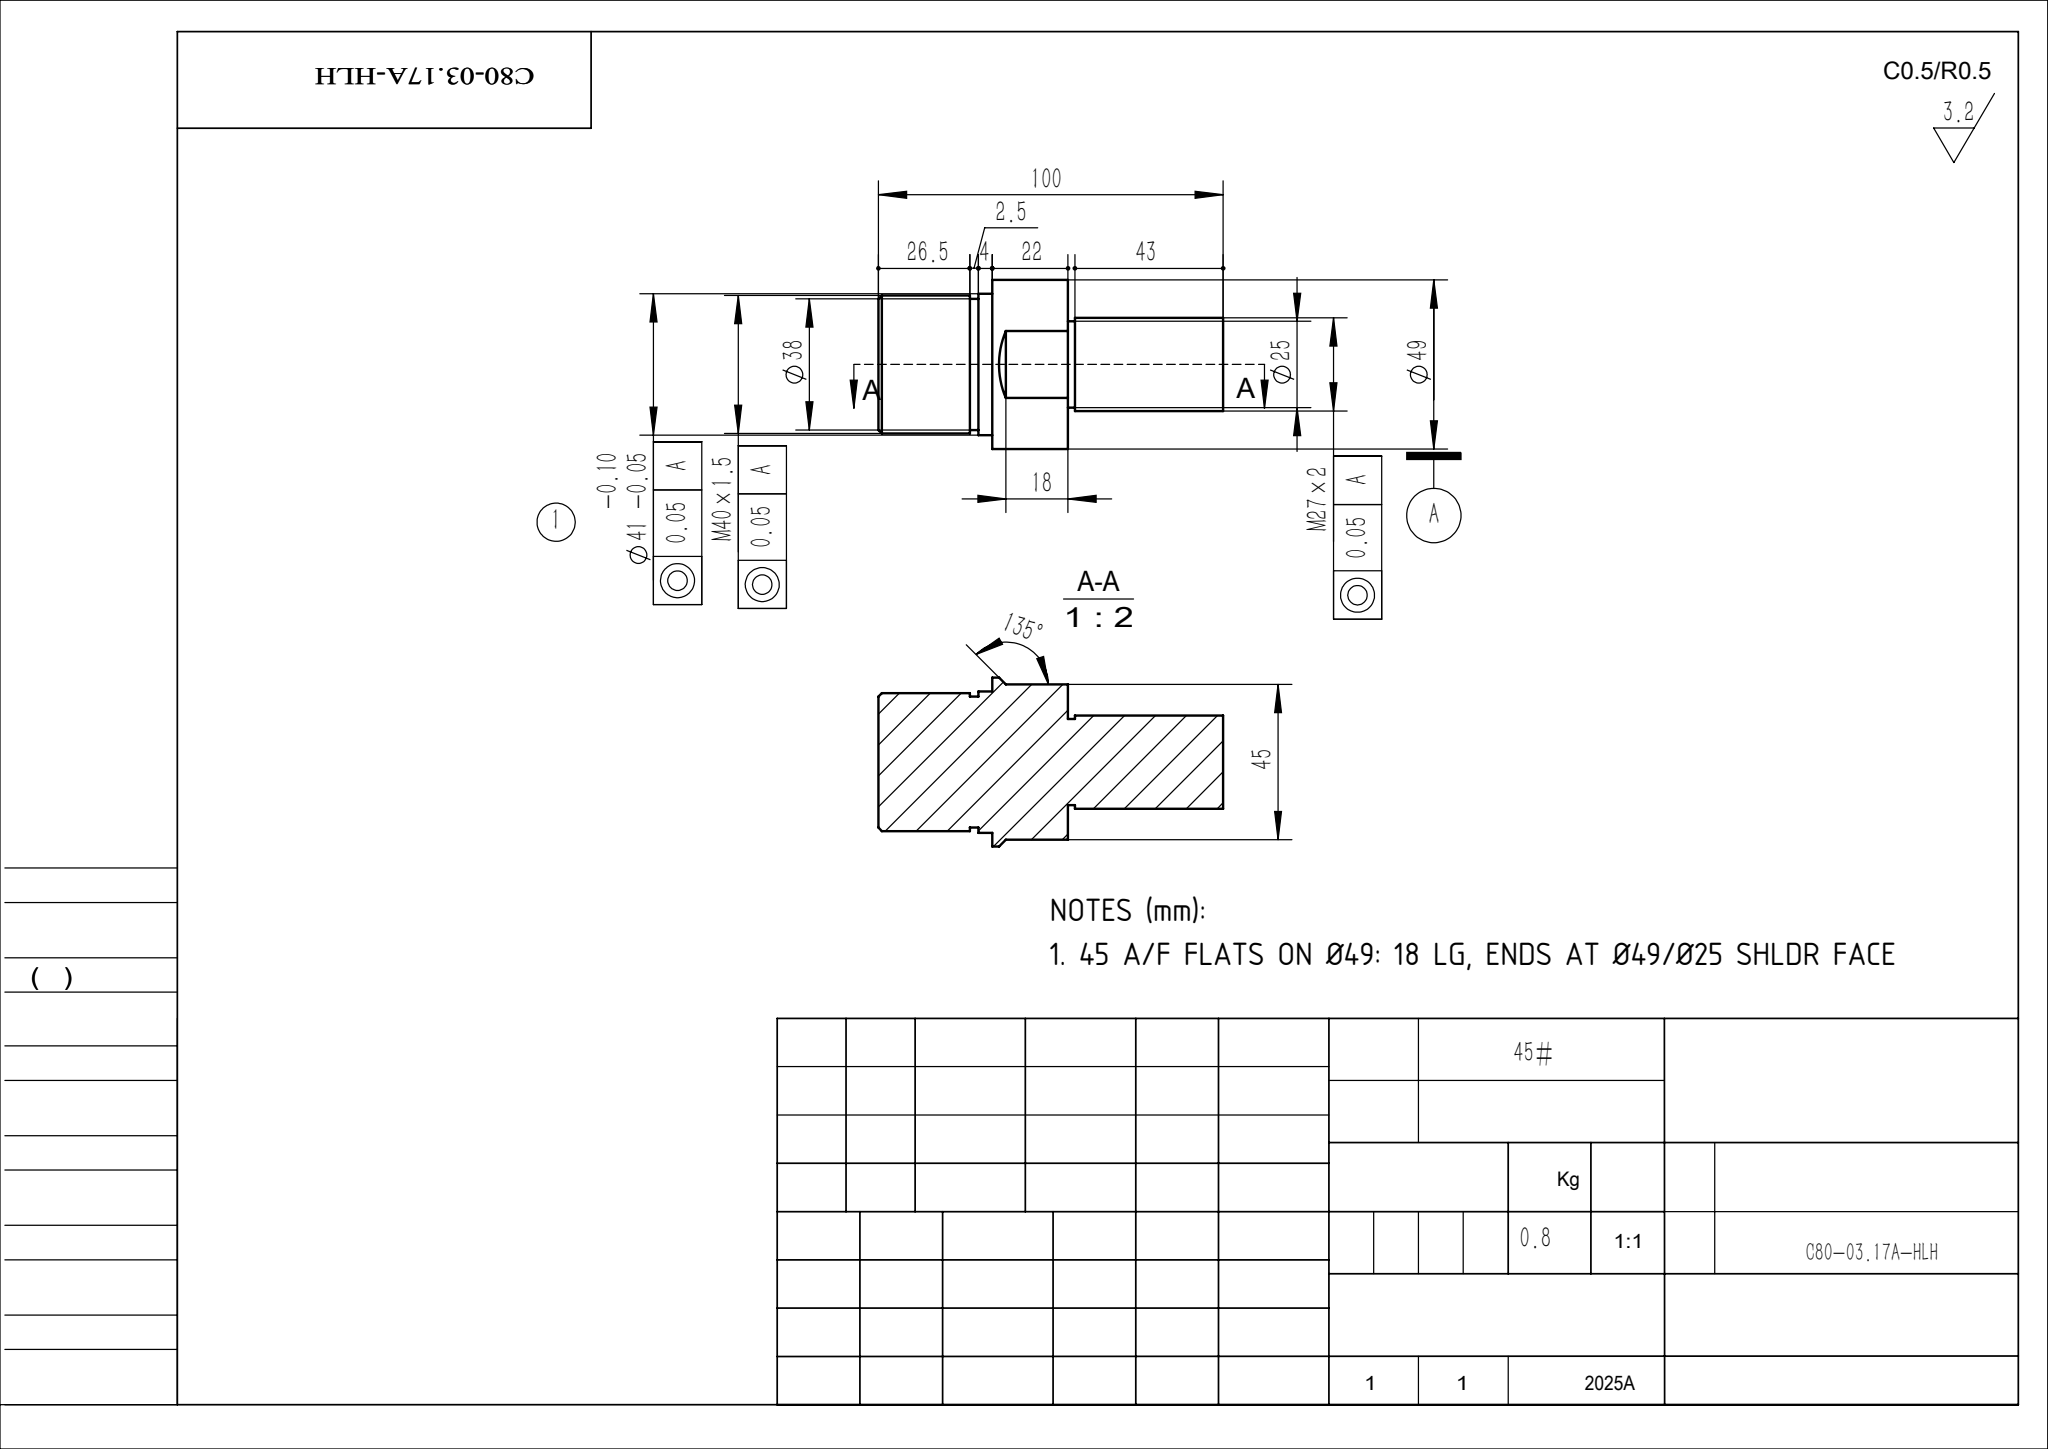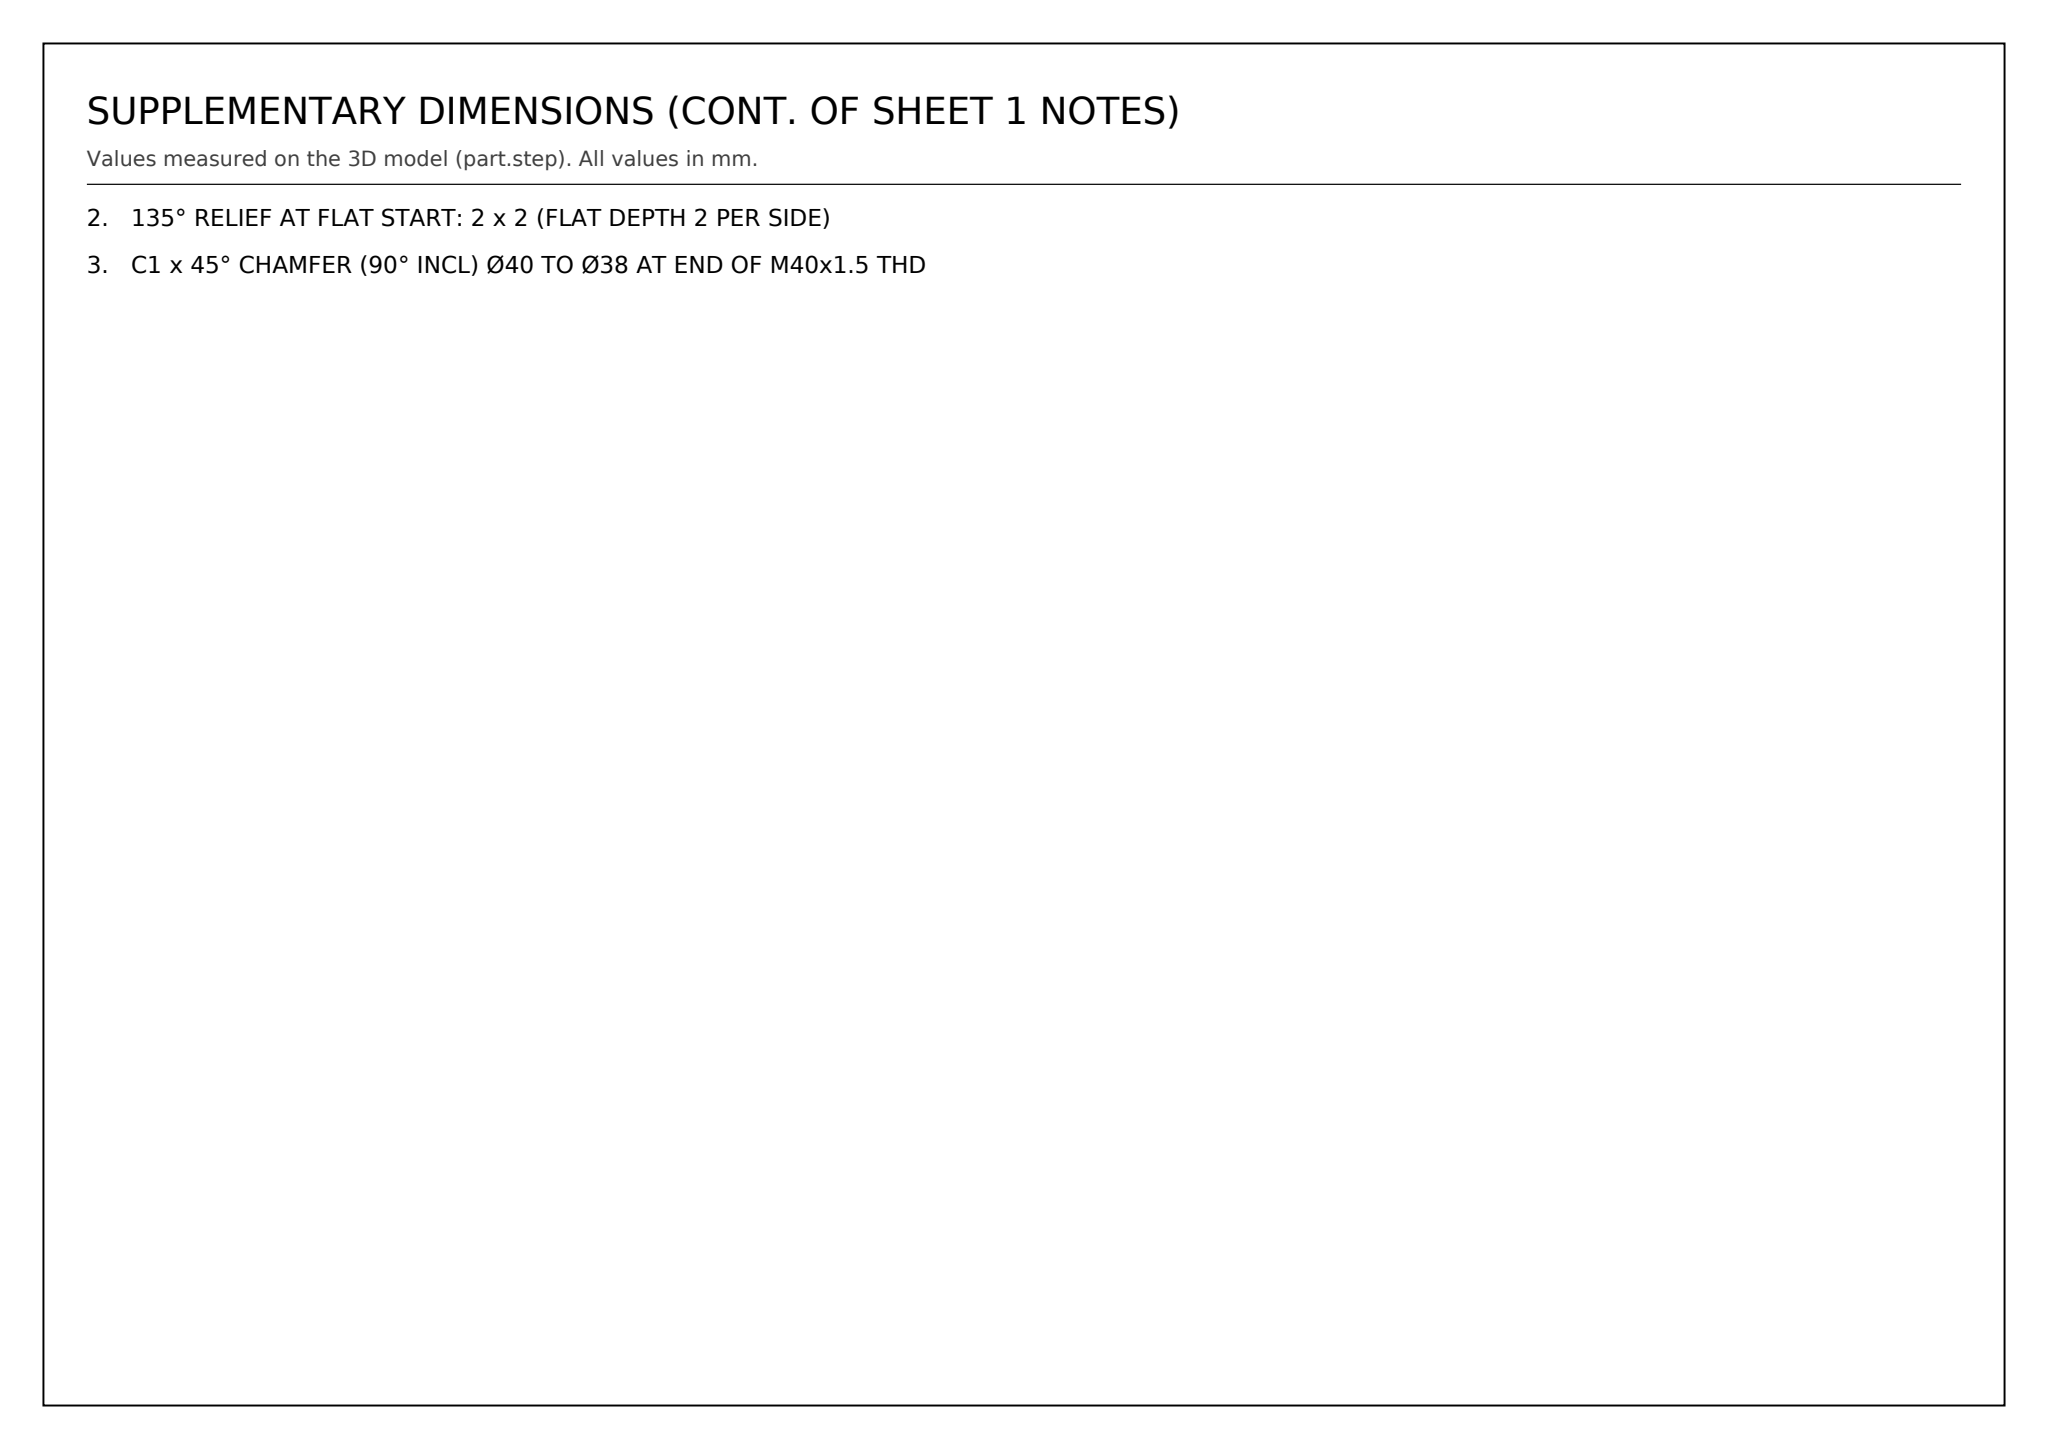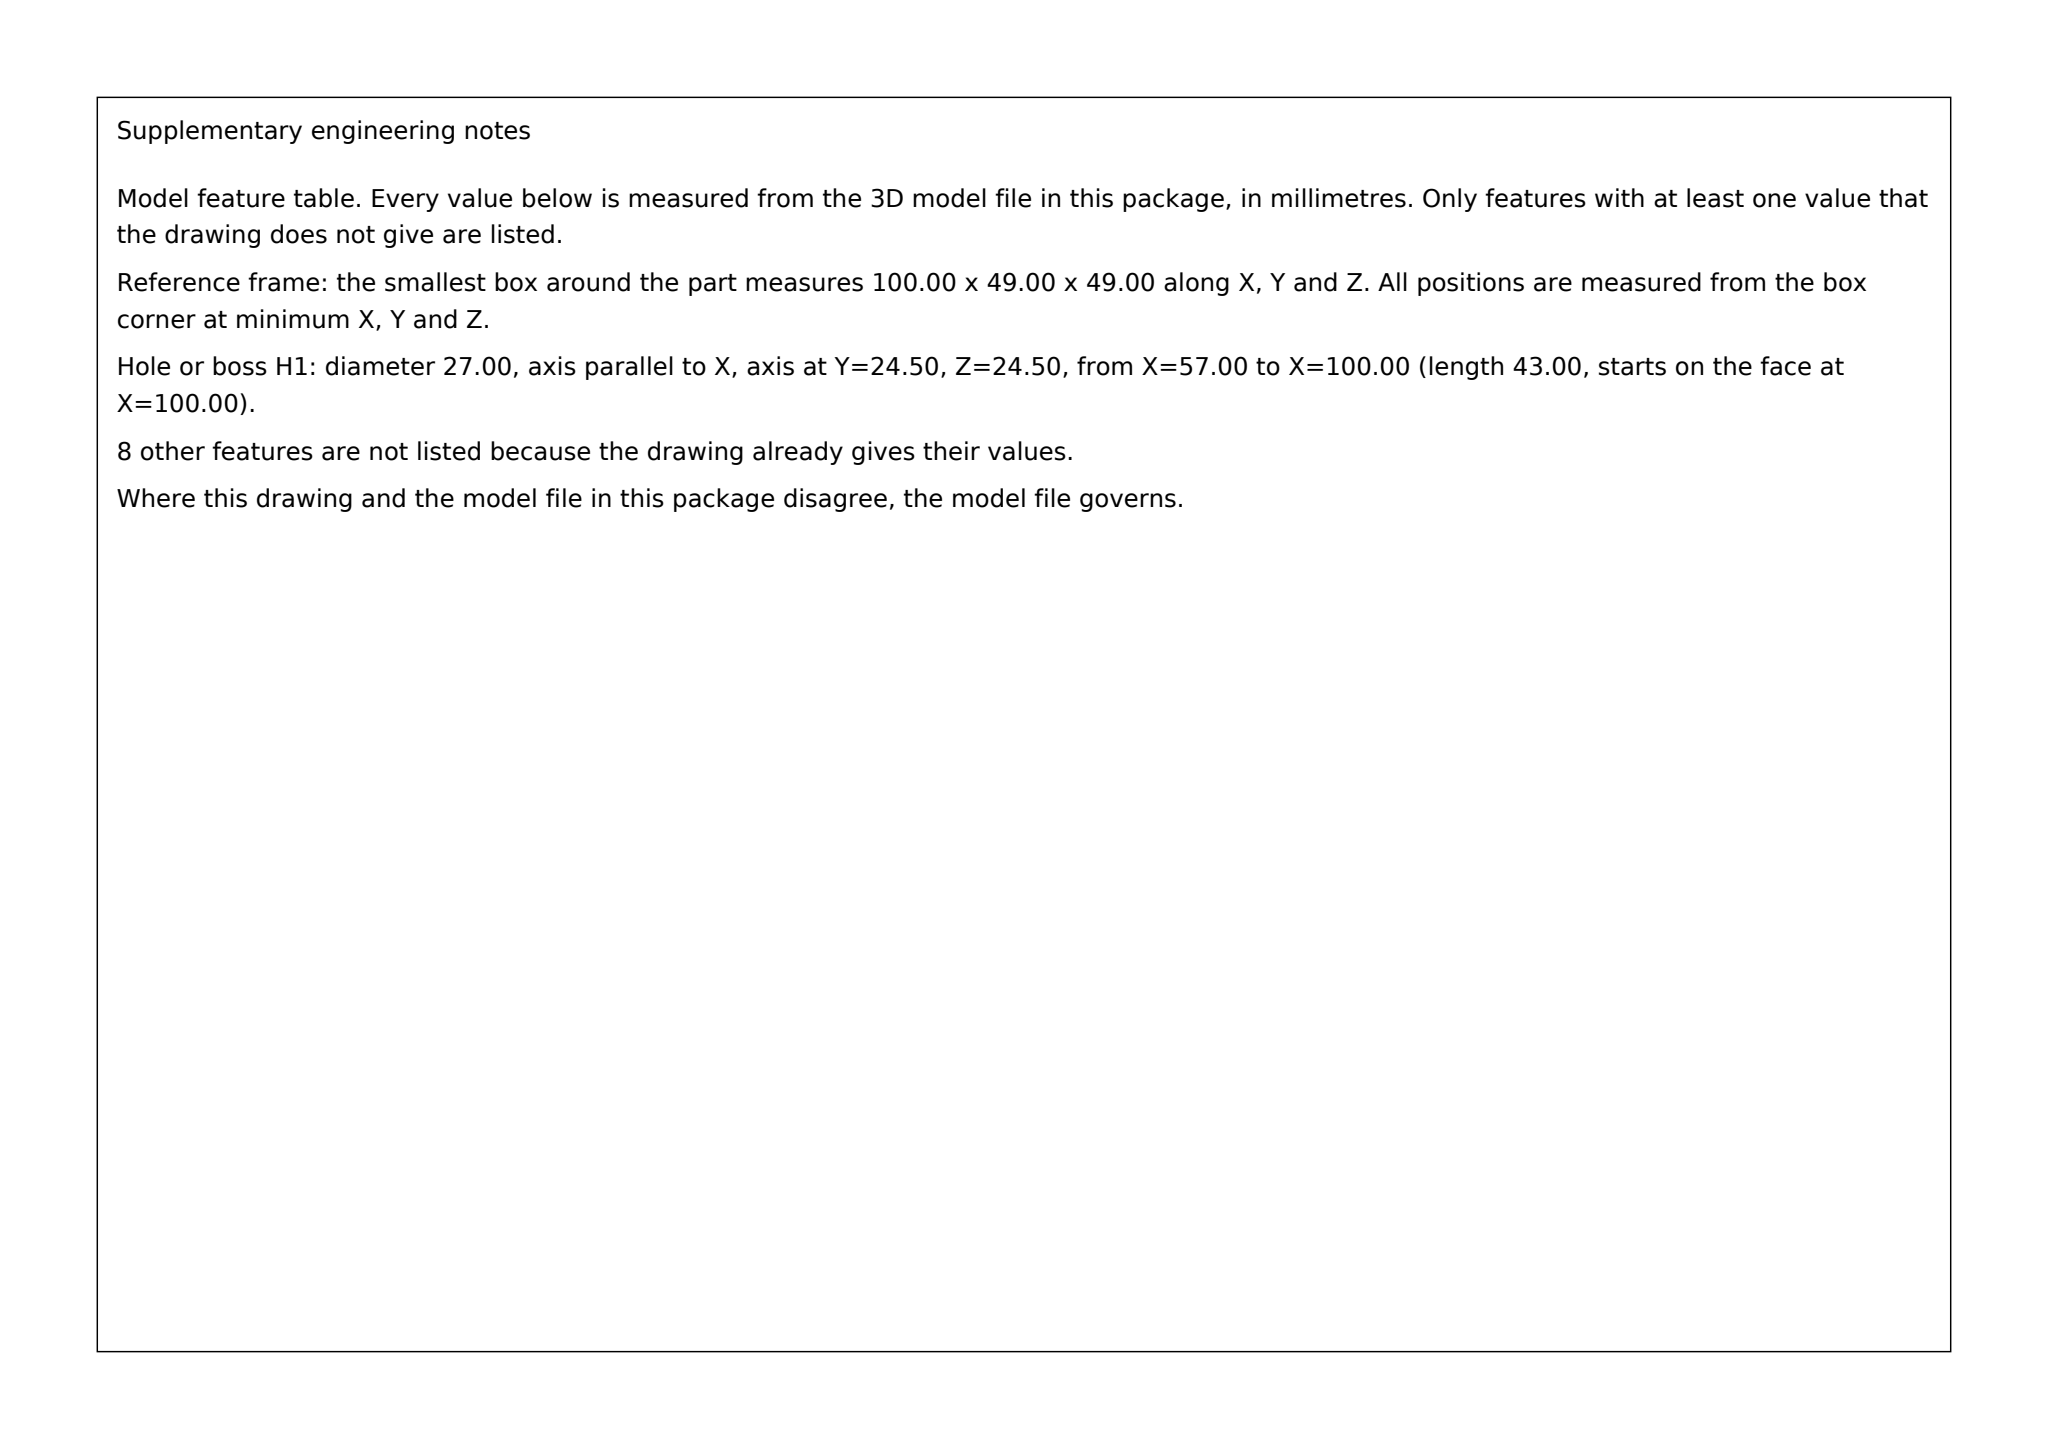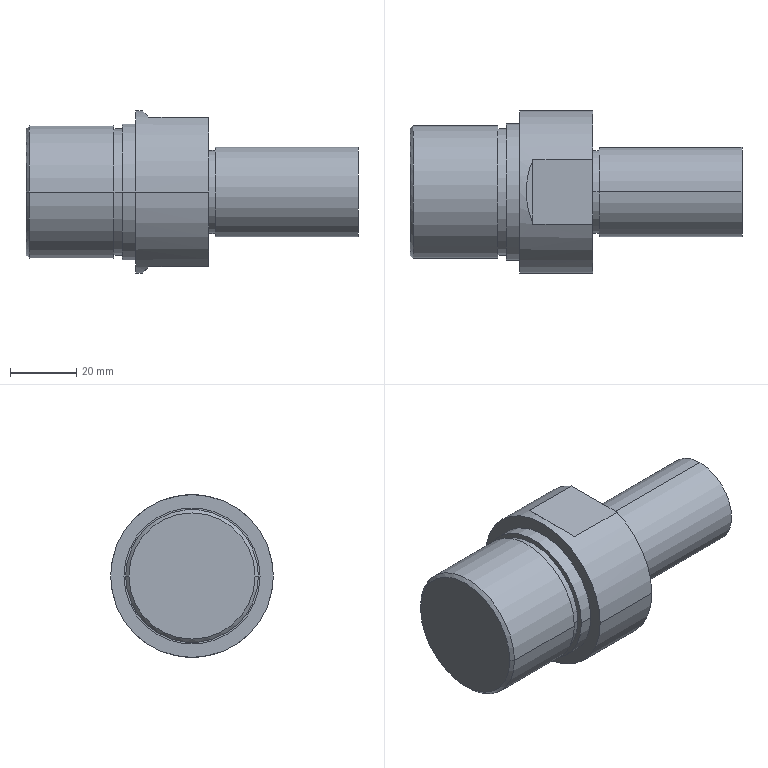Part | SolidWorks | mm | 1 solid | 25 faces | box 100 x 49 x 49 mm | volume 107463 mm3 | cylinder 12 | plane 11 | cone 2 | commonest cylinder face diameters 27 x2 25 x2 49 x2 41 x2 38 x2 40 x2
Drawing notes:
45 A/F FLATS ON Ø49: 18 LG, ENDS AT Ø49/Ø25 SHLDR FACE | from the solid: Flats = planes z=2.49 & 47.49, 45 apart about axis z=24.99 (depth 2 per side on Ø49); Ø49 head spans x=33 to 55 (22 lg); Ø49/Ø25 shoulder = plane x=55, Ø25 undercut 55-57
135° RELIEF AT FLAT START: 2 x 2 (FLAT DEPTH 2 PER SIDE) | from the solid: Ø49 cyl R24.5 to flat at 22.5 from axis (z=2.49/47.49) gives 2 deep; 135° incl. angle = 45° ramp, so 2 axial leg
C1 x 45° CHAMFER (90° INCL) Ø40 TO Ø38 AT END OF M40x1.5 THD | from the solid: cones[90.0 incl, ref_dia 40]; Ø40 cyl L=25.5 ends at x=25.5, plane x=26.5 starts Ø38 undercut → 1 mm axial x 1 mm radial = C1
STEP:
#1=CARTESIAN_POINT('',(87.,0.,-13.5));
#2=VERTEX_POINT('',#1);
#3=CARTESIAN_POINT('',(87.,0.,13.5));
#4=VERTEX_POINT('',#3);
#5=CARTESIAN_POINT('',(87.,0.,0.));
#6=DIRECTION('',(1.,0.,0.));
#7=DIRECTION('',(0.,0.,-1.));
#8=AXIS2_PLACEMENT_3D('',#5,#6,#7);
#9=CIRCLE('',#8,13.5);
#10=EDGE_CURVE('',#2,#4,#9,.T.);
#11=ORIENTED_EDGE('',*,*,#10,.F.);
#12=CARTESIAN_POINT('',(44.,0.,-13.5));
#13=VERTEX_POINT('',#12);
#14=CARTESIAN_POINT('',(87.,0.,-13.5));
#15=DIRECTION('',(-1.,0.,0.));
#16=VECTOR('',#15,1000.);
#17=LINE('',#14,#16);
#18=EDGE_CURVE('',#2,#13,#17,.T.);
#19=ORIENTED_EDGE('',*,*,#18,.T.);
#20=CARTESIAN_POINT('',(44.,0.,13.5));
#21=VERTEX_POINT('',#20);
#22=CARTESIAN_POINT('',(44.,0.,0.));
#23=DIRECTION('',(1.,0.,0.));
#24=DIRECTION('',(0.,0.,-1.));
#25=AXIS2_PLACEMENT_3D('',#22,#23,#24);
#26=CIRCLE('',#25,13.5);
#27=EDGE_CURVE('',#13,#21,#26,.T.);
#28=ORIENTED_EDGE('',*,*,#27,.T.);
#29=CARTESIAN_POINT('',(87.,0.,13.5));
#30=DIRECTION('',(-1.,0.,0.));
#31=VECTOR('',#30,1000.);
#32=LINE('',#29,#31);
#33=EDGE_CURVE('',#4,#21,#32,.T.);
#34=ORIENTED_EDGE('',*,*,#33,.F.);
#35=EDGE_LOOP('',(#11,#19,#28,#34));
#36=FACE_OUTER_BOUND('',#35,.T.);
#37=CARTESIAN_POINT('',(87.,0.,0.));
#38=DIRECTION('',(-1.,0.,0.));
#39=DIRECTION('',(0.,0.,1.));
#40=AXIS2_PLACEMENT_3D('',#37,#38,#39);
#41=CYLINDRICAL_SURFACE('',#40,13.5);
#42=ADVANCED_FACE('',(#36),#41,.T.);
#43=CARTESIAN_POINT('',(44.,0.,-12.5));
#44=VERTEX_POINT('',#43);
#45=CARTESIAN_POINT('',(44.,0.,12.5));
#46=VERTEX_POINT('',#45);
#47=CARTESIAN_POINT('',(44.,0.,0.));
#48=DIRECTION('',(1.,0.,0.));
#49=DIRECTION('',(0.,0.,-1.));
#50=AXIS2_PLACEMENT_3D('',#47,#48,#49);
#51=CIRCLE('',#50,12.5);
#52=EDGE_CURVE('',#44,#46,#51,.T.);
#53=ORIENTED_EDGE('',*,*,#52,.F.);
#54=CARTESIAN_POINT('',(42.,0.,-12.5));
#55=VERTEX_POINT('',#54);
#56=CARTESIAN_POINT('',(44.,0.,-12.5));
#57=DIRECTION('',(-1.,0.,0.));
#58=VECTOR('',#57,1000.);
#59=LINE('',#56,#58);
#60=EDGE_CURVE('',#44,#55,#59,.T.);
#61=ORIENTED_EDGE('',*,*,#60,.T.);
#62=CARTESIAN_POINT('',(42.,0.,12.5));
#63=VERTEX_POINT('',#62);
#64=CARTESIAN_POINT('',(42.,0.,0.));
#65=DIRECTION('',(1.,0.,0.));
#66=DIRECTION('',(0.,0.,-1.));
#67=AXIS2_PLACEMENT_3D('',#64,#65,#66);
#68=CIRCLE('',#67,12.5);
#69=EDGE_CURVE('',#55,#63,#68,.T.);
#70=ORIENTED_EDGE('',*,*,#69,.T.);
#71=CARTESIAN_POINT('',(44.,0.,12.5));
#72=DIRECTION('',(-1.,0.,0.));
#73=VECTOR('',#72,1000.);
#74=LINE('',#71,#73);
#75=EDGE_CURVE('',#46,#63,#74,.T.);
#76=ORIENTED_EDGE('',*,*,#75,.F.);
#77=EDGE_LOOP('',(#53,#61,#70,#76));
#78=FACE_OUTER_BOUND('',#77,.T.);
#79=CARTESIAN_POINT('',(44.,0.,0.));
#80=DIRECTION('',(-1.,0.,0.));
#81=DIRECTION('',(0.,0.,1.));
#82=AXIS2_PLACEMENT_3D('',#79,#80,#81);
#83=CYLINDRICAL_SURFACE('',#82,12.5);
#84=ADVANCED_FACE('',(#78),#83,.T.);
#85=CARTESIAN_POINT('',(42.,24.5,0.));
#86=VERTEX_POINT('',#85);
#87=CARTESIAN_POINT('',(42.,9.695,22.5));
#88=VERTEX_POINT('',#87);
#89=CARTESIAN_POINT('',(42.,-0.,0.));
#90=DIRECTION('',(1.,-0.,0.));
#91=DIRECTION('',(-0.,-1.,0.));
#92=AXIS2_PLACEMENT_3D('',#89,#90,#91);
#93=CIRCLE('',#92,24.5);
#94=EDGE_CURVE('',#86,#88,#93,.T.);
#95=ORIENTED_EDGE('',*,*,#94,.F.);
#96=CARTESIAN_POINT('',(20.,24.5,0.));
#97=VERTEX_POINT('',#96);
#98=CARTESIAN_POINT('',(42.,24.5,0.));
#99=DIRECTION('',(-1.,0.,0.));
#100=VECTOR('',#99,1000.);
#101=LINE('',#98,#100);
#102=EDGE_CURVE('',#86,#97,#101,.T.);
#103=ORIENTED_EDGE('',*,*,#102,.T.);
#104=CARTESIAN_POINT('',(20.,-24.5,0.));
#105=VERTEX_POINT('',#104);
#106=CARTESIAN_POINT('',(20.,0.,0.));
#107=DIRECTION('',(1.,-0.,0.));
#108=DIRECTION('',(-0.,-1.,0.));
#109=AXIS2_PLACEMENT_3D('',#106,#107,#108);
#110=CIRCLE('',#109,24.5);
#111=EDGE_CURVE('',#97,#105,#110,.T.);
#112=ORIENTED_EDGE('',*,*,#111,.T.);
#113=CARTESIAN_POINT('',(42.,-24.5,0.));
#114=VERTEX_POINT('',#113);
#115=CARTESIAN_POINT('',(42.,-24.5,0.));
#116=DIRECTION('',(-1.,0.,0.));
#117=VECTOR('',#116,1000.);
#118=LINE('',#115,#117);
#119=EDGE_CURVE('',#114,#105,#118,.T.);
#120=ORIENTED_EDGE('',*,*,#119,.F.);
#121=CARTESIAN_POINT('',(42.,-9.695,22.5));
#122=VERTEX_POINT('',#121);
#123=CARTESIAN_POINT('',(42.,-0.,0.));
#124=DIRECTION('',(1.,-0.,0.));
#125=DIRECTION('',(-0.,-1.,-0.));
#126=AXIS2_PLACEMENT_3D('',#123,#124,#125);
#127=CIRCLE('',#126,24.5);
#128=EDGE_CURVE('',#122,#114,#127,.T.);
#129=ORIENTED_EDGE('',*,*,#128,.F.);
#130=CARTESIAN_POINT('',(24.,-9.695,22.5));
#131=VERTEX_POINT('',#130);
#132=CARTESIAN_POINT('',(42.,-9.695,22.5));
#133=DIRECTION('',(-1.,0.,0.));
#134=VECTOR('',#133,1000.);
#135=LINE('',#132,#134);
#136=EDGE_CURVE('',#122,#131,#135,.T.);
#137=ORIENTED_EDGE('',*,*,#136,.T.);
#138=CARTESIAN_POINT('',(24.,9.695,22.5));
#139=VERTEX_POINT('',#138);
#140=CARTESIAN_POINT('',(24.,-9.695,22.5));
#141=CARTESIAN_POINT('',(21.295,-3.418,25.205));
#142=CARTESIAN_POINT('',(21.295,3.418,25.205));
#143=CARTESIAN_POINT('',(24.,9.695,22.5));
#144=(BOUNDED_CURVE()B_SPLINE_CURVE(3,(#140,#141,#142,#143),.UNSPECIFIED.,.F.,.F.)B_SPLINE_CURVE_WITH_KNOTS((4,4),(5.876,6.69),.UNSPECIFIED.)CURVE()GEOMETRIC_REPRESENTATION_ITEM()RATIONAL_B_SPLINE_CURVE((1.,0.9456,0.9456,1.))REPRESENTATION_ITEM(''));
#145=EDGE_CURVE('',#131,#139,#144,.T.);
#146=ORIENTED_EDGE('',*,*,#145,.T.);
#147=CARTESIAN_POINT('',(42.,9.695,22.5));
#148=DIRECTION('',(1.,-0.,0.));
#149=VECTOR('',#148,1000.);
#150=LINE('',#147,#149);
#151=EDGE_CURVE('',#139,#88,#150,.T.);
#152=ORIENTED_EDGE('',*,*,#151,.T.);
#153=EDGE_LOOP('',(#95,#103,#112,#120,#129,#137,#146,#152));
#154=FACE_OUTER_BOUND('',#153,.T.);
#155=CARTESIAN_POINT('',(42.,-0.,0.));
#156=DIRECTION('',(-1.,0.,0.));
#157=DIRECTION('',(-0.,-1.,0.));
#158=AXIS2_PLACEMENT_3D('',#155,#156,#157);
#159=CYLINDRICAL_SURFACE('',#158,24.5);
#160=ADVANCED_FACE('',(#154),#159,.T.);
#161=CARTESIAN_POINT('',(16.,20.5,0.));
#162=VERTEX_POINT('',#161);
#163=CARTESIAN_POINT('',(16.,-20.5,0.));
#164=VERTEX_POINT('',#163);
#165=CARTESIAN_POINT('',(16.,-0.,0.));
#166=DIRECTION('',(1.,-0.,0.));
#167=DIRECTION('',(0.,1.,0.));
#168=AXIS2_PLACEMENT_3D('',#165,#166,#167);
#169=CIRCLE('',#168,20.5);
#170=EDGE_CURVE('',#162,#164,#169,.T.);
#171=ORIENTED_EDGE('',*,*,#170,.T.);
#172=CARTESIAN_POINT('',(20.,-20.5,0.));
#173=VERTEX_POINT('',#172);
#174=CARTESIAN_POINT('',(16.,-20.5,0.));
#175=DIRECTION('',(1.,-0.,0.));
#176=VECTOR('',#175,1000.);
#177=LINE('',#174,#176);
#178=EDGE_CURVE('',#164,#173,#177,.T.);
#179=ORIENTED_EDGE('',*,*,#178,.T.);
#180=CARTESIAN_POINT('',(20.,20.5,0.));
#181=VERTEX_POINT('',#180);
#182=CARTESIAN_POINT('',(20.,-0.,0.));
#183=DIRECTION('',(1.,-0.,0.));
#184=DIRECTION('',(0.,1.,0.));
#185=AXIS2_PLACEMENT_3D('',#182,#183,#184);
#186=CIRCLE('',#185,20.5);
#187=EDGE_CURVE('',#181,#173,#186,.T.);
#188=ORIENTED_EDGE('',*,*,#187,.F.);
#189=CARTESIAN_POINT('',(16.,20.5,0.));
#190=DIRECTION('',(1.,-0.,0.));
#191=VECTOR('',#190,1000.);
#192=LINE('',#189,#191);
#193=EDGE_CURVE('',#162,#181,#192,.T.);
#194=ORIENTED_EDGE('',*,*,#193,.F.);
#195=EDGE_LOOP('',(#171,#179,#188,#194));
#196=FACE_OUTER_BOUND('',#195,.T.);
#197=CARTESIAN_POINT('',(16.,-0.,0.));
#198=DIRECTION('',(1.,-0.,0.));
#199=DIRECTION('',(0.,1.,0.));
#200=AXIS2_PLACEMENT_3D('',#197,#198,#199);
#201=CYLINDRICAL_SURFACE('',#200,20.5);
#202=ADVANCED_FACE('',(#196),#201,.T.);
#203=CARTESIAN_POINT('',(13.5,19.,0.));
#204=VERTEX_POINT('',#203);
#205=CARTESIAN_POINT('',(13.5,-19.,0.));
#206=VERTEX_POINT('',#205);
#207=CARTESIAN_POINT('',(13.5,-0.,0.));
#208=DIRECTION('',(1.,-0.,0.));
#209=DIRECTION('',(0.,1.,0.));
#210=AXIS2_PLACEMENT_3D('',#207,#208,#209);
#211=CIRCLE('',#210,19.);
#212=EDGE_CURVE('',#204,#206,#211,.T.);
#213=ORIENTED_EDGE('',*,*,#212,.T.);
#214=CARTESIAN_POINT('',(16.,-19.,0.));
#215=VERTEX_POINT('',#214);
#216=CARTESIAN_POINT('',(13.5,-19.,0.));
#217=DIRECTION('',(1.,-0.,0.));
#218=VECTOR('',#217,1000.);
#219=LINE('',#216,#218);
#220=EDGE_CURVE('',#206,#215,#219,.T.);
#221=ORIENTED_EDGE('',*,*,#220,.T.);
#222=CARTESIAN_POINT('',(16.,19.,0.));
#223=VERTEX_POINT('',#222);
#224=CARTESIAN_POINT('',(16.,-0.,0.));
#225=DIRECTION('',(1.,-0.,0.));
#226=DIRECTION('',(0.,1.,0.));
#227=AXIS2_PLACEMENT_3D('',#224,#225,#226);
#228=CIRCLE('',#227,19.);
#229=EDGE_CURVE('',#223,#215,#228,.T.);
#230=ORIENTED_EDGE('',*,*,#229,.F.);
#231=CARTESIAN_POINT('',(13.5,19.,0.));
#232=DIRECTION('',(1.,-0.,0.));
#233=VECTOR('',#232,1000.);
#234=LINE('',#231,#233);
#235=EDGE_CURVE('',#204,#223,#234,.T.);
#236=ORIENTED_EDGE('',*,*,#235,.F.);
#237=EDGE_LOOP('',(#213,#221,#230,#236));
#238=FACE_OUTER_BOUND('',#237,.T.);
#239=CARTESIAN_POINT('',(13.5,-0.,0.));
#240=DIRECTION('',(1.,-0.,0.));
#241=DIRECTION('',(0.,1.,0.));
#242=AXIS2_PLACEMENT_3D('',#239,#240,#241);
#243=CYLINDRICAL_SURFACE('',#242,19.);
#244=ADVANCED_FACE('',(#238),#243,.T.);
#245=CARTESIAN_POINT('',(-12.,20.,0.));
#246=VERTEX_POINT('',#245);
#247=CARTESIAN_POINT('',(-12.,-20.,0.));
#248=VERTEX_POINT('',#247);
#249=CARTESIAN_POINT('',(-12.,-0.,0.));
#250=DIRECTION('',(1.,0.,0.));
#251=DIRECTION('',(-0.,1.,0.));
#252=AXIS2_PLACEMENT_3D('',#249,#250,#251);
#253=CIRCLE('',#252,20.);
#254=EDGE_CURVE('',#246,#248,#253,.T.);
#255=ORIENTED_EDGE('',*,*,#254,.T.);
#256=CARTESIAN_POINT('',(13.5,-20.,0.));
#257=VERTEX_POINT('',#256);
#258=CARTESIAN_POINT('',(9.5,-20.,0.));
#259=DIRECTION('',(1.,0.,0.));
#260=VECTOR('',#259,1000.);
#261=LINE('',#258,#260);
#262=EDGE_CURVE('',#248,#257,#261,.T.);
#263=ORIENTED_EDGE('',*,*,#262,.T.);
#264=CARTESIAN_POINT('',(13.5,20.,0.));
#265=VERTEX_POINT('',#264);
#266=CARTESIAN_POINT('',(13.5,0.,0.));
#267=DIRECTION('',(-1.,-0.,0.));
#268=DIRECTION('',(-0.,1.,0.));
#269=AXIS2_PLACEMENT_3D('',#266,#267,#268);
#270=CIRCLE('',#269,20.);
#271=EDGE_CURVE('',#257,#265,#270,.T.);
#272=ORIENTED_EDGE('',*,*,#271,.T.);
#273=CARTESIAN_POINT('',(9.5,20.,0.));
#274=DIRECTION('',(1.,0.,0.));
#275=VECTOR('',#274,1000.);
#276=LINE('',#273,#275);
#277=EDGE_CURVE('',#246,#265,#276,.T.);
#278=ORIENTED_EDGE('',*,*,#277,.F.);
#279=EDGE_LOOP('',(#255,#263,#272,#278));
#280=FACE_OUTER_BOUND('',#279,.T.);
#281=CARTESIAN_POINT('',(9.5,0.,0.));
#282=DIRECTION('',(1.,0.,0.));
#283=DIRECTION('',(-0.,1.,0.));
#284=AXIS2_PLACEMENT_3D('',#281,#282,#283);
#285=CYLINDRICAL_SURFACE('',#284,20.);
#286=ADVANCED_FACE('',(#280),#285,.T.);
#287=CARTESIAN_POINT('',(-13.,19.,0.));
#288=VERTEX_POINT('',#287);
#289=CARTESIAN_POINT('',(-13.,-19.,0.));
#290=VERTEX_POINT('',#289);
#291=CARTESIAN_POINT('',(-13.,-0.,0.));
#292=DIRECTION('',(1.,0.,-0.));
#293=DIRECTION('',(-0.,1.,0.));
#294=AXIS2_PLACEMENT_3D('',#291,#292,#293);
#295=CIRCLE('',#294,19.);
#296=EDGE_CURVE('',#288,#290,#295,.T.);
#297=ORIENTED_EDGE('',*,*,#296,.T.);
#298=CARTESIAN_POINT('',(-12.,-20.,0.));
#299=DIRECTION('',(0.7071,-0.7071,0.));
#300=VECTOR('',#299,1000.);
#301=LINE('',#298,#300);
#302=EDGE_CURVE('',#290,#248,#301,.T.);
#303=ORIENTED_EDGE('',*,*,#302,.T.);
#304=ORIENTED_EDGE('',*,*,#254,.F.);
#305=CARTESIAN_POINT('',(-12.,20.,-0.));
#306=DIRECTION('',(0.7071,0.7071,-0.));
#307=VECTOR('',#306,1000.);
#308=LINE('',#305,#307);
#309=EDGE_CURVE('',#288,#246,#308,.T.);
#310=ORIENTED_EDGE('',*,*,#309,.F.);
#311=EDGE_LOOP('',(#297,#303,#304,#310));
#312=FACE_OUTER_BOUND('',#311,.T.);
#313=CARTESIAN_POINT('',(-12.,-0.,-0.));
#314=DIRECTION('',(1.,0.,-0.));
#315=DIRECTION('',(-0.,1.,0.));
#316=AXIS2_PLACEMENT_3D('',#313,#314,#315);
#317=CONICAL_SURFACE('',#316,20.,0.7854);
#318=ADVANCED_FACE('',(#312),#317,.T.);
#319=CARTESIAN_POINT('',(42.,0.,0.));
#320=DIRECTION('',(1.,0.,0.));
#321=DIRECTION('',(0.,0.,-1.));
#322=AXIS2_PLACEMENT_3D('',#319,#320,#321);
#323=CIRCLE('',#322,12.5);
#324=EDGE_CURVE('',#63,#55,#323,.T.);
#325=ORIENTED_EDGE('',*,*,#324,.F.);
#326=ORIENTED_EDGE('',*,*,#69,.F.);
#327=EDGE_LOOP('',(#325,#326));
#328=FACE_BOUND('',#327,.T.);
#329=CARTESIAN_POINT('',(42.,21.5,22.5));
#330=DIRECTION('',(0.,-1.,0.));
#331=VECTOR('',#330,1000.);
#332=LINE('',#329,#331);
#333=EDGE_CURVE('',#88,#122,#332,.T.);
#334=ORIENTED_EDGE('',*,*,#333,.T.);
#335=ORIENTED_EDGE('',*,*,#128,.T.);
#336=CARTESIAN_POINT('',(42.,-9.695,-22.5));
#337=VERTEX_POINT('',#336);
#338=CARTESIAN_POINT('',(42.,-0.,0.));
#339=DIRECTION('',(1.,-0.,0.));
#340=DIRECTION('',(-0.,-1.,0.));
#341=AXIS2_PLACEMENT_3D('',#338,#339,#340);
#342=CIRCLE('',#341,24.5);
#343=EDGE_CURVE('',#114,#337,#342,.T.);
#344=ORIENTED_EDGE('',*,*,#343,.T.);
#345=CARTESIAN_POINT('',(42.,9.695,-22.5));
#346=VERTEX_POINT('',#345);
#347=CARTESIAN_POINT('',(42.,21.5,-22.5));
#348=DIRECTION('',(0.,1.,0.));
#349=VECTOR('',#348,1000.);
#350=LINE('',#347,#349);
#351=EDGE_CURVE('',#337,#346,#350,.T.);
#352=ORIENTED_EDGE('',*,*,#351,.T.);
#353=CARTESIAN_POINT('',(42.,-0.,0.));
#354=DIRECTION('',(1.,-0.,0.));
#355=DIRECTION('',(-0.,-1.,0.));
#356=AXIS2_PLACEMENT_3D('',#353,#354,#355);
#357=CIRCLE('',#356,24.5);
#358=EDGE_CURVE('',#346,#86,#357,.T.);
#359=ORIENTED_EDGE('',*,*,#358,.T.);
#360=ORIENTED_EDGE('',*,*,#94,.T.);
#361=EDGE_LOOP('',(#334,#335,#344,#352,#359,#360));
#362=FACE_OUTER_BOUND('',#361,.T.);
#363=CARTESIAN_POINT('',(42.,21.5,0.));
#364=DIRECTION('',(1.,0.,0.));
#365=DIRECTION('',(0.,0.,-1.));
#366=AXIS2_PLACEMENT_3D('',#363,#364,#365);
#367=PLANE('',#366);
#368=ADVANCED_FACE('',(#328,#362),#367,.T.);
#369=ORIENTED_EDGE('',*,*,#102,.F.);
#370=ORIENTED_EDGE('',*,*,#358,.F.);
#371=CARTESIAN_POINT('',(24.,9.695,-22.5));
#372=VERTEX_POINT('',#371);
#373=CARTESIAN_POINT('',(42.,9.695,-22.5));
#374=DIRECTION('',(-1.,0.,0.));
#375=VECTOR('',#374,1000.);
#376=LINE('',#373,#375);
#377=EDGE_CURVE('',#346,#372,#376,.T.);
#378=ORIENTED_EDGE('',*,*,#377,.T.);
#379=CARTESIAN_POINT('',(24.,-9.695,-22.5));
#380=VERTEX_POINT('',#379);
#381=CARTESIAN_POINT('',(24.,9.695,-22.5));
#382=CARTESIAN_POINT('',(21.295,3.418,-25.205));
#383=CARTESIAN_POINT('',(21.295,-3.418,-25.205));
#384=CARTESIAN_POINT('',(24.,-9.695,-22.5));
#385=(BOUNDED_CURVE()B_SPLINE_CURVE(3,(#381,#382,#383,#384),.UNSPECIFIED.,.F.,.T.)B_SPLINE_CURVE_WITH_KNOTS((4,4),(5.876,6.69),.UNSPECIFIED.)CURVE()GEOMETRIC_REPRESENTATION_ITEM()RATIONAL_B_SPLINE_CURVE((1.,0.9456,0.9456,1.))REPRESENTATION_ITEM(''));
#386=EDGE_CURVE('',#372,#380,#385,.T.);
#387=ORIENTED_EDGE('',*,*,#386,.T.);
#388=CARTESIAN_POINT('',(42.,-9.695,-22.5));
#389=DIRECTION('',(1.,-0.,0.));
#390=VECTOR('',#389,1000.);
#391=LINE('',#388,#390);
#392=EDGE_CURVE('',#380,#337,#391,.T.);
#393=ORIENTED_EDGE('',*,*,#392,.T.);
#394=ORIENTED_EDGE('',*,*,#343,.F.);
#395=ORIENTED_EDGE('',*,*,#119,.T.);
#396=CARTESIAN_POINT('',(20.,0.,0.));
#397=DIRECTION('',(1.,-0.,0.));
#398=DIRECTION('',(-0.,-1.,0.));
#399=AXIS2_PLACEMENT_3D('',#396,#397,#398);
#400=CIRCLE('',#399,24.5);
#401=EDGE_CURVE('',#105,#97,#400,.T.);
#402=ORIENTED_EDGE('',*,*,#401,.T.);
#403=EDGE_LOOP('',(#369,#370,#378,#387,#393,#394,#395,#402));
#404=FACE_OUTER_BOUND('',#403,.T.);
#405=CARTESIAN_POINT('',(42.,-0.,0.));
#406=DIRECTION('',(-1.,0.,0.));
#407=DIRECTION('',(-0.,-1.,0.));
#408=AXIS2_PLACEMENT_3D('',#405,#406,#407);
#409=CYLINDRICAL_SURFACE('',#408,24.5);
#410=ADVANCED_FACE('',(#404),#409,.T.);
#411=ORIENTED_EDGE('',*,*,#333,.F.);
#412=ORIENTED_EDGE('',*,*,#151,.F.);
#413=CARTESIAN_POINT('',(24.,0.,22.5));
#414=DIRECTION('',(0.,1.,0.));
#415=VECTOR('',#414,1000.);
#416=LINE('',#413,#415);
#417=EDGE_CURVE('',#131,#139,#416,.T.);
#418=ORIENTED_EDGE('',*,*,#417,.F.);
#419=ORIENTED_EDGE('',*,*,#136,.F.);
#420=EDGE_LOOP('',(#411,#412,#418,#419));
#421=FACE_OUTER_BOUND('',#420,.T.);
#422=CARTESIAN_POINT('',(42.,0.,22.5));
#423=DIRECTION('',(0.,0.,-1.));
#424=DIRECTION('',(-1.,0.,0.));
#425=AXIS2_PLACEMENT_3D('',#422,#423,#424);
#426=PLANE('',#425);
#427=ADVANCED_FACE('',(#421),#426,.F.);
#428=ORIENTED_EDGE('',*,*,#351,.F.);
#429=ORIENTED_EDGE('',*,*,#392,.F.);
#430=CARTESIAN_POINT('',(24.,0.,-22.5));
#431=DIRECTION('',(0.,-1.,0.));
#432=VECTOR('',#431,1000.);
#433=LINE('',#430,#432);
#434=EDGE_CURVE('',#372,#380,#433,.T.);
#435=ORIENTED_EDGE('',*,*,#434,.F.);
#436=ORIENTED_EDGE('',*,*,#377,.F.);
#437=EDGE_LOOP('',(#428,#429,#435,#436));
#438=FACE_OUTER_BOUND('',#437,.T.);
#439=CARTESIAN_POINT('',(42.,0.,-22.5));
#440=DIRECTION('',(0.,0.,1.));
#441=DIRECTION('',(1.,0.,0.));
#442=AXIS2_PLACEMENT_3D('',#439,#440,#441);
#443=PLANE('',#442);
#444=ADVANCED_FACE('',(#438),#443,.F.);
#445=ORIENTED_EDGE('',*,*,#187,.T.);
#446=CARTESIAN_POINT('',(20.,-0.,0.));
#447=DIRECTION('',(1.,-0.,0.));
#448=DIRECTION('',(0.,1.,0.));
#449=AXIS2_PLACEMENT_3D('',#446,#447,#448);
#450=CIRCLE('',#449,20.5);
#451=EDGE_CURVE('',#173,#181,#450,.T.);
#452=ORIENTED_EDGE('',*,*,#451,.T.);
#453=EDGE_LOOP('',(#445,#452));
#454=FACE_BOUND('',#453,.T.);
#455=ORIENTED_EDGE('',*,*,#401,.F.);
#456=ORIENTED_EDGE('',*,*,#111,.F.);
#457=EDGE_LOOP('',(#455,#456));
#458=FACE_OUTER_BOUND('',#457,.T.);
#459=CARTESIAN_POINT('',(20.,22.5,0.));
#460=DIRECTION('',(-1.,0.,0.));
#461=DIRECTION('',(-0.,-1.,0.));
#462=AXIS2_PLACEMENT_3D('',#459,#460,#461);
#463=PLANE('',#462);
#464=ADVANCED_FACE('',(#454,#458),#463,.T.);
#465=ORIENTED_EDGE('',*,*,#434,.T.);
#466=ORIENTED_EDGE('',*,*,#386,.F.);
#467=EDGE_LOOP('',(#465,#466));
#468=FACE_OUTER_BOUND('',#467,.T.);
#469=CARTESIAN_POINT('',(24.,0.,-22.5));
#470=DIRECTION('',(0.7071,0.,-0.7071));
#471=DIRECTION('',(-0.7071,0.,-0.7071));
#472=AXIS2_PLACEMENT_3D('',#469,#470,#471);
#473=PLANE('',#472);
#474=ADVANCED_FACE('',(#468),#473,.T.);
#475=ORIENTED_EDGE('',*,*,#417,.T.);
#476=ORIENTED_EDGE('',*,*,#145,.F.);
#477=EDGE_LOOP('',(#475,#476));
#478=FACE_OUTER_BOUND('',#477,.T.);
#479=CARTESIAN_POINT('',(24.,0.,22.5));
#480=DIRECTION('',(0.7071,0.,0.7071));
#481=DIRECTION('',(0.7071,0.,-0.7071));
#482=AXIS2_PLACEMENT_3D('',#479,#480,#481);
#483=PLANE('',#482);
#484=ADVANCED_FACE('',(#478),#483,.T.);
#485=ORIENTED_EDGE('',*,*,#178,.F.);
#486=CARTESIAN_POINT('',(16.,-0.,0.));
#487=DIRECTION('',(1.,-0.,0.));
#488=DIRECTION('',(0.,1.,0.));
#489=AXIS2_PLACEMENT_3D('',#486,#487,#488);
#490=CIRCLE('',#489,20.5);
#491=EDGE_CURVE('',#164,#162,#490,.T.);
#492=ORIENTED_EDGE('',*,*,#491,.T.);
#493=ORIENTED_EDGE('',*,*,#193,.T.);
#494=ORIENTED_EDGE('',*,*,#451,.F.);
#495=EDGE_LOOP('',(#485,#492,#493,#494));
#496=FACE_OUTER_BOUND('',#495,.T.);
#497=CARTESIAN_POINT('',(16.,-0.,0.));
#498=DIRECTION('',(1.,-0.,0.));
#499=DIRECTION('',(0.,1.,0.));
#500=AXIS2_PLACEMENT_3D('',#497,#498,#499);
#501=CYLINDRICAL_SURFACE('',#500,20.5);
#502=ADVANCED_FACE('',(#496),#501,.T.);
#503=ORIENTED_EDGE('',*,*,#229,.T.);
#504=CARTESIAN_POINT('',(16.,-0.,0.));
#505=DIRECTION('',(1.,-0.,0.));
#506=DIRECTION('',(0.,1.,0.));
#507=AXIS2_PLACEMENT_3D('',#504,#505,#506);
#508=CIRCLE('',#507,19.);
#509=EDGE_CURVE('',#215,#223,#508,.T.);
#510=ORIENTED_EDGE('',*,*,#509,.T.);
#511=EDGE_LOOP('',(#503,#510));
#512=FACE_BOUND('',#511,.T.);
#513=ORIENTED_EDGE('',*,*,#170,.F.);
#514=ORIENTED_EDGE('',*,*,#491,.F.);
#515=EDGE_LOOP('',(#513,#514));
#516=FACE_OUTER_BOUND('',#515,.T.);
#517=CARTESIAN_POINT('',(16.,-0.,0.));
#518=DIRECTION('',(-1.,0.,0.));
#519=DIRECTION('',(-0.,-1.,0.));
#520=AXIS2_PLACEMENT_3D('',#517,#518,#519);
#521=PLANE('',#520);
#522=ADVANCED_FACE('',(#512,#516),#521,.T.);
#523=ORIENTED_EDGE('',*,*,#220,.F.);
#524=CARTESIAN_POINT('',(13.5,-0.,0.));
#525=DIRECTION('',(1.,-0.,0.));
#526=DIRECTION('',(0.,1.,0.));
#527=AXIS2_PLACEMENT_3D('',#524,#525,#526);
#528=CIRCLE('',#527,19.);
#529=EDGE_CURVE('',#206,#204,#528,.T.);
#530=ORIENTED_EDGE('',*,*,#529,.T.);
#531=ORIENTED_EDGE('',*,*,#235,.T.);
#532=ORIENTED_EDGE('',*,*,#509,.F.);
#533=EDGE_LOOP('',(#523,#530,#531,#532));
#534=FACE_OUTER_BOUND('',#533,.T.);
#535=CARTESIAN_POINT('',(13.5,-0.,0.));
#536=DIRECTION('',(1.,-0.,0.));
#537=DIRECTION('',(0.,1.,0.));
#538=AXIS2_PLACEMENT_3D('',#535,#536,#537);
#539=CYLINDRICAL_SURFACE('',#538,19.);
#540=ADVANCED_FACE('',(#534),#539,.T.);
#541=ORIENTED_EDGE('',*,*,#212,.F.);
#542=ORIENTED_EDGE('',*,*,#529,.F.);
#543=EDGE_LOOP('',(#541,#542));
#544=FACE_BOUND('',#543,.T.);
#545=CARTESIAN_POINT('',(13.5,0.,0.));
#546=DIRECTION('',(-1.,-0.,0.));
#547=DIRECTION('',(-0.,1.,0.));
#548=AXIS2_PLACEMENT_3D('',#545,#546,#547);
#549=CIRCLE('',#548,20.);
#550=EDGE_CURVE('',#265,#257,#549,.T.);
#551=ORIENTED_EDGE('',*,*,#550,.F.);
#552=ORIENTED_EDGE('',*,*,#271,.F.);
#553=EDGE_LOOP('',(#551,#552));
#554=FACE_OUTER_BOUND('',#553,.T.);
#555=CARTESIAN_POINT('',(13.5,-0.,0.));
#556=DIRECTION('',(-1.,0.,0.));
#557=DIRECTION('',(-0.,-1.,0.));
#558=AXIS2_PLACEMENT_3D('',#555,#556,#557);
#559=PLANE('',#558);
#560=ADVANCED_FACE('',(#544,#554),#559,.F.);
#561=ORIENTED_EDGE('',*,*,#262,.F.);
#562=CARTESIAN_POINT('',(-12.,-0.,0.));
#563=DIRECTION('',(1.,0.,0.));
#564=DIRECTION('',(-0.,1.,0.));
#565=AXIS2_PLACEMENT_3D('',#562,#563,#564);
#566=CIRCLE('',#565,20.);
#567=EDGE_CURVE('',#248,#246,#566,.T.);
#568=ORIENTED_EDGE('',*,*,#567,.T.);
#569=ORIENTED_EDGE('',*,*,#277,.T.);
#570=ORIENTED_EDGE('',*,*,#550,.T.);
#571=EDGE_LOOP('',(#561,#568,#569,#570));
#572=FACE_OUTER_BOUND('',#571,.T.);
#573=CARTESIAN_POINT('',(9.5,0.,0.));
#574=DIRECTION('',(1.,0.,0.));
#575=DIRECTION('',(-0.,1.,0.));
#576=AXIS2_PLACEMENT_3D('',#573,#574,#575);
#577=CYLINDRICAL_SURFACE('',#576,20.);
#578=ADVANCED_FACE('',(#572),#577,.T.);
#579=ORIENTED_EDGE('',*,*,#302,.F.);
#580=CARTESIAN_POINT('',(-13.,-0.,0.));
#581=DIRECTION('',(1.,0.,-0.));
#582=DIRECTION('',(-0.,1.,0.));
#583=AXIS2_PLACEMENT_3D('',#580,#581,#582);
#584=CIRCLE('',#583,19.);
#585=EDGE_CURVE('',#290,#288,#584,.T.);
#586=ORIENTED_EDGE('',*,*,#585,.T.);
#587=ORIENTED_EDGE('',*,*,#309,.T.);
#588=ORIENTED_EDGE('',*,*,#567,.F.);
#589=EDGE_LOOP('',(#579,#586,#587,#588));
#590=FACE_OUTER_BOUND('',#589,.T.);
#591=CARTESIAN_POINT('',(-12.,-0.,-0.));
#592=DIRECTION('',(1.,0.,-0.));
#593=DIRECTION('',(-0.,1.,0.));
#594=AXIS2_PLACEMENT_3D('',#591,#592,#593);
#595=CONICAL_SURFACE('',#594,20.,0.7854);
#596=ADVANCED_FACE('',(#590),#595,.T.);
#597=ORIENTED_EDGE('',*,*,#296,.F.);
#598=ORIENTED_EDGE('',*,*,#585,.F.);
#599=EDGE_LOOP('',(#597,#598));
#600=FACE_OUTER_BOUND('',#599,.T.);
#601=CARTESIAN_POINT('',(-13.,0.,0.));
#602=DIRECTION('',(1.,-0.,0.));
#603=DIRECTION('',(0.,1.,0.));
#604=AXIS2_PLACEMENT_3D('',#601,#602,#603);
#605=PLANE('',#604);
#606=ADVANCED_FACE('',(#600),#605,.F.);
#607=ORIENTED_EDGE('',*,*,#60,.F.);
#608=CARTESIAN_POINT('',(44.,0.,0.));
#609=DIRECTION('',(1.,0.,0.));
#610=DIRECTION('',(0.,0.,-1.));
#611=AXIS2_PLACEMENT_3D('',#608,#609,#610);
#612=CIRCLE('',#611,12.5);
#613=EDGE_CURVE('',#46,#44,#612,.T.);
#614=ORIENTED_EDGE('',*,*,#613,.F.);
#615=ORIENTED_EDGE('',*,*,#75,.T.);
#616=ORIENTED_EDGE('',*,*,#324,.T.);
#617=EDGE_LOOP('',(#607,#614,#615,#616));
#618=FACE_OUTER_BOUND('',#617,.T.);
#619=CARTESIAN_POINT('',(44.,0.,0.));
#620=DIRECTION('',(-1.,0.,0.));
#621=DIRECTION('',(0.,0.,1.));
#622=AXIS2_PLACEMENT_3D('',#619,#620,#621);
#623=CYLINDRICAL_SURFACE('',#622,12.5);
#624=ADVANCED_FACE('',(#618),#623,.T.);
#625=ORIENTED_EDGE('',*,*,#18,.F.);
#626=CARTESIAN_POINT('',(87.,0.,0.));
#627=DIRECTION('',(1.,0.,0.));
#628=DIRECTION('',(0.,0.,-1.));
#629=AXIS2_PLACEMENT_3D('',#626,#627,#628);
#630=CIRCLE('',#629,13.5);
#631=EDGE_CURVE('',#4,#2,#630,.T.);
#632=ORIENTED_EDGE('',*,*,#631,.F.);
#633=ORIENTED_EDGE('',*,*,#33,.T.);
#634=CARTESIAN_POINT('',(44.,0.,0.));
#635=DIRECTION('',(1.,0.,0.));
#636=DIRECTION('',(0.,0.,-1.));
#637=AXIS2_PLACEMENT_3D('',#634,#635,#636);
#638=CIRCLE('',#637,13.5);
#639=EDGE_CURVE('',#21,#13,#638,.T.);
#640=ORIENTED_EDGE('',*,*,#639,.T.);
#641=EDGE_LOOP('',(#625,#632,#633,#640));
#642=FACE_OUTER_BOUND('',#641,.T.);
#643=CARTESIAN_POINT('',(87.,0.,0.));
#644=DIRECTION('',(-1.,0.,0.));
#645=DIRECTION('',(0.,0.,1.));
#646=AXIS2_PLACEMENT_3D('',#643,#644,#645);
#647=CYLINDRICAL_SURFACE('',#646,13.5);
#648=ADVANCED_FACE('',(#642),#647,.T.);
#649=ORIENTED_EDGE('',*,*,#631,.T.);
#650=ORIENTED_EDGE('',*,*,#10,.T.);
#651=EDGE_LOOP('',(#649,#650));
#652=FACE_OUTER_BOUND('',#651,.T.);
#653=CARTESIAN_POINT('',(87.,0.,0.));
#654=DIRECTION('',(1.,0.,0.));
#655=DIRECTION('',(0.,0.,-1.));
#656=AXIS2_PLACEMENT_3D('',#653,#654,#655);
#657=PLANE('',#656);
#658=ADVANCED_FACE('',(#652),#657,.T.);
#659=ORIENTED_EDGE('',*,*,#613,.T.);
#660=ORIENTED_EDGE('',*,*,#52,.T.);
#661=EDGE_LOOP('',(#659,#660));
#662=FACE_BOUND('',#661,.T.);
#663=ORIENTED_EDGE('',*,*,#639,.F.);
#664=ORIENTED_EDGE('',*,*,#27,.F.);
#665=EDGE_LOOP('',(#663,#664));
#666=FACE_OUTER_BOUND('',#665,.T.);
#667=CARTESIAN_POINT('',(44.,0.,0.));
#668=DIRECTION('',(1.,0.,0.));
#669=DIRECTION('',(0.,0.,-1.));
#670=AXIS2_PLACEMENT_3D('',#667,#668,#669);
#671=PLANE('',#670);
#672=ADVANCED_FACE('',(#662,#666),#671,.F.);
#673=CLOSED_SHELL('',(#42,#84,#160,#202,#244,#286,#318,#368,#410,#427,#444,#464,#474,#484,#502,#522,#540,#560,#578,#596,#606,#624,#648,#658,#672));
#674=MANIFOLD_SOLID_BREP('',#673);
#675=CARTESIAN_POINT('',(0.,0.,0.));
#676=DIRECTION('',(0.,0.,1.));
#677=DIRECTION('',(1.,0.,0.));
#678=AXIS2_PLACEMENT_3D('',#675,#676,#677);
#679=(LENGTH_UNIT()NAMED_UNIT(*)SI_UNIT(.MILLI.,.METRE.));
#680=UNCERTAINTY_MEASURE_WITH_UNIT(LENGTH_MEASURE(0.00001),#679,'','');
#681=(NAMED_UNIT(*)PLANE_ANGLE_UNIT()SI_UNIT($,.RADIAN.));
#682=(NAMED_UNIT(*)SI_UNIT($,.STERADIAN.)SOLID_ANGLE_UNIT());
#683=(GEOMETRIC_REPRESENTATION_CONTEXT(3)GLOBAL_UNCERTAINTY_ASSIGNED_CONTEXT((#680))GLOBAL_UNIT_ASSIGNED_CONTEXT((#679,#681,#682))REPRESENTATION_CONTEXT('',''));
#684=ADVANCED_BREP_SHAPE_REPRESENTATION('',(#674,#678),#683);